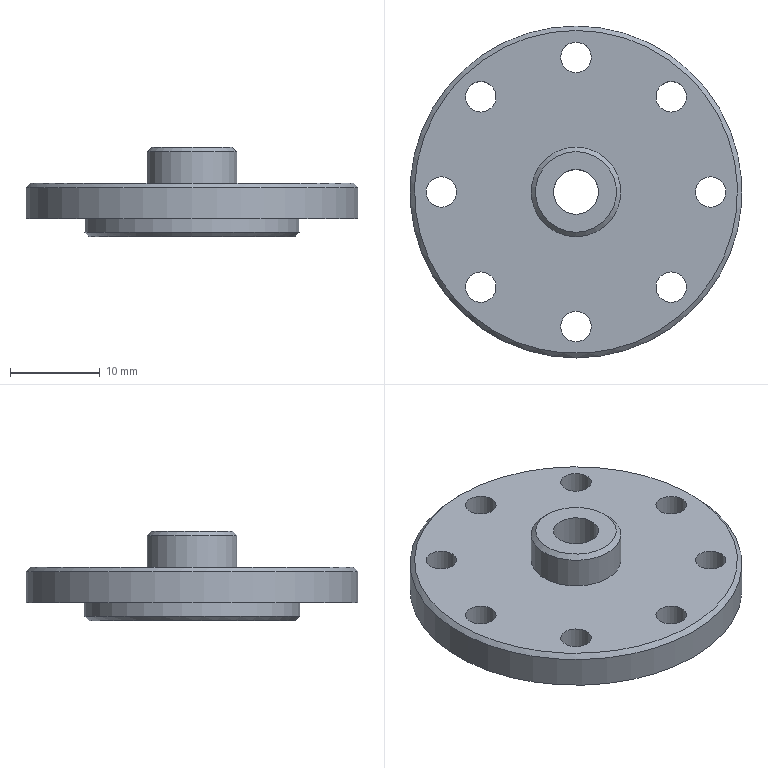Component | NX | CYLINDER_HEAD | 1 solid | 19 faces | volume 5005 mm3 | cylinder 12 | plane 4 | cone 3 | commonest cylinder face diameters 3.4 x8 24 x1 37 x1 10 x1 5 x1